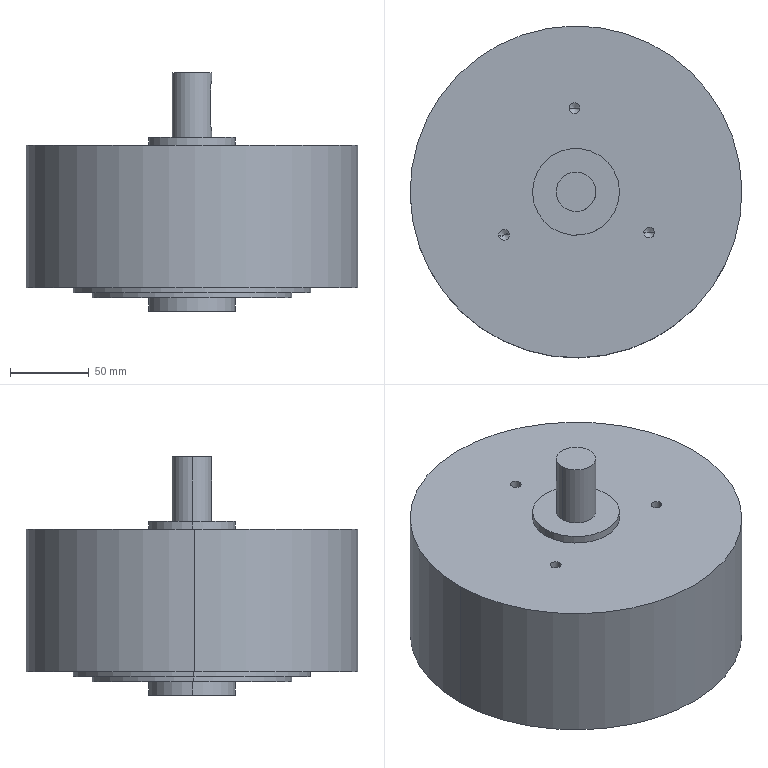Component | SolidWorks | HB-114BHysteresisClutch-1 | 1 solid | 37 faces | box 210 x 210 x 151 mm | volume 3263911 mm3 | cylinder 21 | plane 10 | cone 6 | commonest cylinder face diameters 6.8 x6 55 x4 8 x3 126.361 x2 150.627 x2 210 x2 25 x2 | material A3
build123d program:
from build123d import *

# Parameters (mm, degrees)
CUT_EXTRUDE1_START    = 12.5
CUT_EXTRUDE1_DEPTH    = 4
M8_TAPPED_HOLE1_D     = 6.8
M8_TAPPED_HOLE1_DEPTH = 19.75
M8_TAPPED_HOLE1_TIP   = 2.043


with BuildPart() as part:
    # Sketch1 → Revolve1 (revolve)
    with BuildSketch(Plane.XY, mode=Mode.PRIVATE) as revolve1_sk:
        Polygon((0, 0), (151, 0), (151, 27.5), (142.307, 27.5), (142.307, 63.181), (139.421, 63.181), (139.421, 75.314), (136, 75.314), (136, 105), (46, 105), (46, 27.5), (41, 27.5), (41, 12.5), (0, 12.5), align=None)
    revolve(revolve1_sk.sketch.rotate(Axis((0, 0, 0), (-1, 0, 0)), 90), axis=Axis((0, 0, 0), (-1, 0, 0)))

    # Sketch2 → Cut-Extrude1 (cut)
    with BuildSketch(Plane.XY.offset(CUT_EXTRUDE1_START)):
        with BuildLine():
            Line((9, 4), (33, 4))
            ThreePointArc((33, 4), (37, 0), (33, -4))
            Line((33, -4), (9, -4))
            ThreePointArc((9, -4), (5, 0), (9, 4))
        make_face()
    extrude(amount=-CUT_EXTRUDE1_DEPTH, mode=Mode.SUBTRACT)

    # M8 Tapped Hole1
    with Locations(Plane.ZY.offset(-46)):
        with Locations((0, 53), (45.899, -26.5), (-45.899, -26.5)):
            Hole(M8_TAPPED_HOLE1_D / 2, depth=M8_TAPPED_HOLE1_DEPTH)
            with Locations((0, 0, -(M8_TAPPED_HOLE1_DEPTH + M8_TAPPED_HOLE1_TIP / 2))):  # 118° drill point
                Cone(0, M8_TAPPED_HOLE1_D / 2, M8_TAPPED_HOLE1_TIP, mode=Mode.SUBTRACT)


solid = part.part

# Placed as in the assembly
solid = solid.moved(Location((733.029, 200.722, -58.5), (-90, 89.057, 90)))
STEP:
#1=CARTESIAN_POINT('',(28.691,9.987,-4.892));
#2=VERTEX_POINT('',#1);
#3=CARTESIAN_POINT('',(28.959,9.991,-4.892));
#4=VERTEX_POINT('',#3);
#5=CARTESIAN_POINT('',(28.825,9.989,-4.892));
#6=DIRECTION('',(-0.,-0.,1.));
#7=DIRECTION('',(0.9999,0.01645,0.));
#8=AXIS2_PLACEMENT_3D('',#5,#6,#7);
#9=CIRCLE('',#8,0.1339);
#10=EDGE_CURVE('',#2,#4,#9,.T.);
#11=ORIENTED_EDGE('',*,*,#10,.F.);
#12=CARTESIAN_POINT('',(28.691,9.987,-4.114));
#13=VERTEX_POINT('',#12);
#14=CARTESIAN_POINT('',(28.691,9.987,-4.114));
#15=DIRECTION('',(-0.,-0.,1.));
#16=VECTOR('',#15,39.37);
#17=LINE('',#14,#16);
#18=EDGE_CURVE('',#2,#13,#17,.T.);
#19=ORIENTED_EDGE('',*,*,#18,.T.);
#20=CARTESIAN_POINT('',(28.959,9.991,-4.114));
#21=VERTEX_POINT('',#20);
#22=CARTESIAN_POINT('',(28.825,9.989,-4.114));
#23=DIRECTION('',(-0.,-0.,1.));
#24=DIRECTION('',(0.9999,0.01645,0.));
#25=AXIS2_PLACEMENT_3D('',#22,#23,#24);
#26=CIRCLE('',#25,0.1339);
#27=EDGE_CURVE('',#13,#21,#26,.T.);
#28=ORIENTED_EDGE('',*,*,#27,.T.);
#29=CARTESIAN_POINT('',(28.959,9.991,-4.114));
#30=DIRECTION('',(-0.,-0.,1.));
#31=VECTOR('',#30,39.37);
#32=LINE('',#29,#31);
#33=EDGE_CURVE('',#4,#21,#32,.T.);
#34=ORIENTED_EDGE('',*,*,#33,.F.);
#35=EDGE_LOOP('',(#11,#19,#28,#34));
#36=FACE_OUTER_BOUND('',#35,.T.);
#37=CARTESIAN_POINT('',(28.825,9.989,-4.114));
#38=DIRECTION('',(-0.,-0.,1.));
#39=DIRECTION('',(0.9999,0.01645,0.));
#40=AXIS2_PLACEMENT_3D('',#37,#38,#39);
#41=CYLINDRICAL_SURFACE('',#40,0.1339);
#42=ADVANCED_FACE('',(#36),#41,.F.);
#43=CARTESIAN_POINT('',(28.825,9.989,-4.972));
#44=VERTEX_POINT('',#43);
#45=CARTESIAN_POINT('',(28.959,9.991,-4.892));
#46=DIRECTION('',(0.8571,0.0141,0.515));
#47=VECTOR('',#46,39.37);
#48=LINE('',#45,#47);
#49=EDGE_CURVE('',#44,#4,#48,.T.);
#50=ORIENTED_EDGE('',*,*,#49,.F.);
#51=CARTESIAN_POINT('',(28.691,9.987,-4.892));
#52=DIRECTION('',(-0.8571,-0.0141,0.515));
#53=VECTOR('',#52,39.37);
#54=LINE('',#51,#53);
#55=EDGE_CURVE('',#44,#2,#54,.T.);
#56=ORIENTED_EDGE('',*,*,#55,.T.);
#57=ORIENTED_EDGE('',*,*,#10,.T.);
#58=EDGE_LOOP('',(#50,#56,#57));
#59=FACE_OUTER_BOUND('',#58,.T.);
#60=CARTESIAN_POINT('',(28.825,9.989,-4.892));
#61=DIRECTION('',(-0.,-0.,1.));
#62=DIRECTION('',(0.9999,0.01645,0.));
#63=AXIS2_PLACEMENT_3D('',#60,#61,#62);
#64=CONICAL_SURFACE('',#63,0.1339,1.03);
#65=ADVANCED_FACE('',(#59),#64,.F.);
#66=CARTESIAN_POINT('',(30.55,6.887,-4.892));
#67=VERTEX_POINT('',#66);
#68=CARTESIAN_POINT('',(30.817,6.891,-4.892));
#69=VERTEX_POINT('',#68);
#70=CARTESIAN_POINT('',(30.683,6.889,-4.892));
#71=DIRECTION('',(-0.,-0.,1.));
#72=DIRECTION('',(0.9999,0.01645,0.));
#73=AXIS2_PLACEMENT_3D('',#70,#71,#72);
#74=CIRCLE('',#73,0.1339);
#75=EDGE_CURVE('',#67,#69,#74,.T.);
#76=ORIENTED_EDGE('',*,*,#75,.F.);
#77=CARTESIAN_POINT('',(30.55,6.887,-4.114));
#78=VERTEX_POINT('',#77);
#79=CARTESIAN_POINT('',(30.55,6.887,-4.114));
#80=DIRECTION('',(-0.,-0.,1.));
#81=VECTOR('',#80,39.37);
#82=LINE('',#79,#81);
#83=EDGE_CURVE('',#67,#78,#82,.T.);
#84=ORIENTED_EDGE('',*,*,#83,.T.);
#85=CARTESIAN_POINT('',(30.817,6.891,-4.114));
#86=VERTEX_POINT('',#85);
#87=CARTESIAN_POINT('',(30.683,6.889,-4.114));
#88=DIRECTION('',(-0.,-0.,1.));
#89=DIRECTION('',(0.9999,0.01645,0.));
#90=AXIS2_PLACEMENT_3D('',#87,#88,#89);
#91=CIRCLE('',#90,0.1339);
#92=EDGE_CURVE('',#78,#86,#91,.T.);
#93=ORIENTED_EDGE('',*,*,#92,.T.);
#94=CARTESIAN_POINT('',(30.817,6.891,-4.114));
#95=DIRECTION('',(-0.,-0.,1.));
#96=VECTOR('',#95,39.37);
#97=LINE('',#94,#96);
#98=EDGE_CURVE('',#69,#86,#97,.T.);
#99=ORIENTED_EDGE('',*,*,#98,.F.);
#100=EDGE_LOOP('',(#76,#84,#93,#99));
#101=FACE_OUTER_BOUND('',#100,.T.);
#102=CARTESIAN_POINT('',(30.683,6.889,-4.114));
#103=DIRECTION('',(-0.,-0.,1.));
#104=DIRECTION('',(0.9999,0.01645,0.));
#105=AXIS2_PLACEMENT_3D('',#102,#103,#104);
#106=CYLINDRICAL_SURFACE('',#105,0.1339);
#107=ADVANCED_FACE('',(#101),#106,.F.);
#108=CARTESIAN_POINT('',(30.683,6.889,-4.972));
#109=VERTEX_POINT('',#108);
#110=CARTESIAN_POINT('',(30.817,6.891,-4.892));
#111=DIRECTION('',(0.8571,0.0141,0.515));
#112=VECTOR('',#111,39.37);
#113=LINE('',#110,#112);
#114=EDGE_CURVE('',#109,#69,#113,.T.);
#115=ORIENTED_EDGE('',*,*,#114,.F.);
#116=CARTESIAN_POINT('',(30.55,6.887,-4.892));
#117=DIRECTION('',(-0.8571,-0.0141,0.515));
#118=VECTOR('',#117,39.37);
#119=LINE('',#116,#118);
#120=EDGE_CURVE('',#109,#67,#119,.T.);
#121=ORIENTED_EDGE('',*,*,#120,.T.);
#122=ORIENTED_EDGE('',*,*,#75,.T.);
#123=EDGE_LOOP('',(#115,#121,#122));
#124=FACE_OUTER_BOUND('',#123,.T.);
#125=CARTESIAN_POINT('',(30.683,6.889,-4.892));
#126=DIRECTION('',(-0.,-0.,1.));
#127=DIRECTION('',(0.9999,0.01645,0.));
#128=AXIS2_PLACEMENT_3D('',#125,#126,#127);
#129=CONICAL_SURFACE('',#128,0.1339,1.03);
#130=ADVANCED_FACE('',(#124),#129,.F.);
#131=CARTESIAN_POINT('',(26.936,6.827,-4.892));
#132=VERTEX_POINT('',#131);
#133=CARTESIAN_POINT('',(27.204,6.832,-4.892));
#134=VERTEX_POINT('',#133);
#135=CARTESIAN_POINT('',(27.07,6.83,-4.892));
#136=DIRECTION('',(-0.,-0.,1.));
#137=DIRECTION('',(0.9999,0.01645,0.));
#138=AXIS2_PLACEMENT_3D('',#135,#136,#137);
#139=CIRCLE('',#138,0.1339);
#140=EDGE_CURVE('',#132,#134,#139,.T.);
#141=ORIENTED_EDGE('',*,*,#140,.F.);
#142=CARTESIAN_POINT('',(26.936,6.827,-4.114));
#143=VERTEX_POINT('',#142);
#144=CARTESIAN_POINT('',(26.936,6.827,-4.114));
#145=DIRECTION('',(-0.,-0.,1.));
#146=VECTOR('',#145,39.37);
#147=LINE('',#144,#146);
#148=EDGE_CURVE('',#132,#143,#147,.T.);
#149=ORIENTED_EDGE('',*,*,#148,.T.);
#150=CARTESIAN_POINT('',(27.204,6.832,-4.114));
#151=VERTEX_POINT('',#150);
#152=CARTESIAN_POINT('',(27.07,6.83,-4.114));
#153=DIRECTION('',(-0.,-0.,1.));
#154=DIRECTION('',(0.9999,0.01645,0.));
#155=AXIS2_PLACEMENT_3D('',#152,#153,#154);
#156=CIRCLE('',#155,0.1339);
#157=EDGE_CURVE('',#143,#151,#156,.T.);
#158=ORIENTED_EDGE('',*,*,#157,.T.);
#159=CARTESIAN_POINT('',(27.204,6.832,-4.114));
#160=DIRECTION('',(-0.,-0.,1.));
#161=VECTOR('',#160,39.37);
#162=LINE('',#159,#161);
#163=EDGE_CURVE('',#134,#151,#162,.T.);
#164=ORIENTED_EDGE('',*,*,#163,.F.);
#165=EDGE_LOOP('',(#141,#149,#158,#164));
#166=FACE_OUTER_BOUND('',#165,.T.);
#167=CARTESIAN_POINT('',(27.07,6.83,-4.114));
#168=DIRECTION('',(-0.,-0.,1.));
#169=DIRECTION('',(0.9999,0.01645,0.));
#170=AXIS2_PLACEMENT_3D('',#167,#168,#169);
#171=CYLINDRICAL_SURFACE('',#170,0.1339);
#172=ADVANCED_FACE('',(#166),#171,.F.);
#173=CARTESIAN_POINT('',(27.07,6.83,-4.972));
#174=VERTEX_POINT('',#173);
#175=CARTESIAN_POINT('',(27.204,6.832,-4.892));
#176=DIRECTION('',(0.8571,0.0141,0.515));
#177=VECTOR('',#176,39.37);
#178=LINE('',#175,#177);
#179=EDGE_CURVE('',#174,#134,#178,.T.);
#180=ORIENTED_EDGE('',*,*,#179,.F.);
#181=CARTESIAN_POINT('',(26.936,6.827,-4.892));
#182=DIRECTION('',(-0.8571,-0.0141,0.515));
#183=VECTOR('',#182,39.37);
#184=LINE('',#181,#183);
#185=EDGE_CURVE('',#174,#132,#184,.T.);
#186=ORIENTED_EDGE('',*,*,#185,.T.);
#187=ORIENTED_EDGE('',*,*,#140,.T.);
#188=EDGE_LOOP('',(#180,#186,#187));
#189=FACE_OUTER_BOUND('',#188,.T.);
#190=CARTESIAN_POINT('',(27.07,6.83,-4.892));
#191=DIRECTION('',(-0.,-0.,1.));
#192=DIRECTION('',(0.9999,0.01645,0.));
#193=AXIS2_PLACEMENT_3D('',#190,#191,#192);
#194=CONICAL_SURFACE('',#193,0.1339,1.03);
#195=ADVANCED_FACE('',(#189),#194,.F.);
#196=CARTESIAN_POINT('',(29.194,7.908,-3.76));
#197=VERTEX_POINT('',#196);
#198=CARTESIAN_POINT('',(29.191,8.065,-3.602));
#199=VERTEX_POINT('',#198);
#200=CARTESIAN_POINT('',(29.194,7.908,-3.602));
#201=DIRECTION('',(0.9999,0.01645,0.));
#202=DIRECTION('',(0.,0.,-1.));
#203=AXIS2_PLACEMENT_3D('',#200,#201,#202);
#204=CIRCLE('',#203,0.1575);
#205=EDGE_CURVE('',#197,#199,#204,.T.);
#206=ORIENTED_EDGE('',*,*,#205,.F.);
#207=CARTESIAN_POINT('',(29.351,7.911,-3.76));
#208=VERTEX_POINT('',#207);
#209=CARTESIAN_POINT('',(29.194,7.908,-3.76));
#210=DIRECTION('',(0.9999,0.01645,0.));
#211=VECTOR('',#210,39.37);
#212=LINE('',#209,#211);
#213=EDGE_CURVE('',#197,#208,#212,.T.);
#214=ORIENTED_EDGE('',*,*,#213,.T.);
#215=CARTESIAN_POINT('',(29.323,8.068,-3.602));
#216=VERTEX_POINT('',#215);
#217=CARTESIAN_POINT('',(29.351,7.911,-3.76));
#218=CARTESIAN_POINT('',(29.351,7.921,-3.76));
#219=CARTESIAN_POINT('',(29.351,7.931,-3.759));
#220=CARTESIAN_POINT('',(29.349,7.952,-3.755));
#221=CARTESIAN_POINT('',(29.348,7.961,-3.752));
#222=CARTESIAN_POINT('',(29.345,7.981,-3.744));
#223=CARTESIAN_POINT('',(29.344,7.99,-3.739));
#224=CARTESIAN_POINT('',(29.34,8.006,-3.728));
#225=CARTESIAN_POINT('',(29.339,8.014,-3.721));
#226=CARTESIAN_POINT('',(29.335,8.029,-3.706));
#227=CARTESIAN_POINT('',(29.333,8.035,-3.699));
#228=CARTESIAN_POINT('',(29.33,8.047,-3.682));
#229=CARTESIAN_POINT('',(29.328,8.052,-3.672));
#230=CARTESIAN_POINT('',(29.326,8.059,-3.653));
#231=CARTESIAN_POINT('',(29.325,8.062,-3.644));
#232=CARTESIAN_POINT('',(29.323,8.067,-3.623));
#233=CARTESIAN_POINT('',(29.323,8.068,-3.613));
#234=CARTESIAN_POINT('',(29.323,8.068,-3.602));
#235=B_SPLINE_CURVE_WITH_KNOTS('',3,(#217,#218,#219,#220,#221,#222,#223,#224,#225,#226,#227,#228,#229,#230,#231,#232,#233,#234),.UNSPECIFIED.,.F.,.F.,(4,2,2,2,2,2,2,2,4),(0.006296,0.007082,0.007868,0.008654,0.00944,0.01023,0.01101,0.0118,0.01258),.UNSPECIFIED.);
#236=EDGE_CURVE('',#208,#216,#235,.T.);
#237=ORIENTED_EDGE('',*,*,#236,.T.);
#238=CARTESIAN_POINT('',(29.191,8.065,-3.602));
#239=DIRECTION('',(0.9999,0.01645,0.));
#240=VECTOR('',#239,39.37);
#241=LINE('',#238,#240);
#242=EDGE_CURVE('',#199,#216,#241,.T.);
#243=ORIENTED_EDGE('',*,*,#242,.F.);
#244=EDGE_LOOP('',(#206,#214,#237,#243));
#245=FACE_OUTER_BOUND('',#244,.T.);
#246=CARTESIAN_POINT('',(29.194,7.908,-3.602));
#247=DIRECTION('',(0.9999,0.01645,0.));
#248=DIRECTION('',(0.,0.,-1.));
#249=AXIS2_PLACEMENT_3D('',#246,#247,#248);
#250=CYLINDRICAL_SURFACE('',#249,0.1575);
#251=ADVANCED_FACE('',(#245),#250,.F.);
#252=CARTESIAN_POINT('',(26.372,7.862,-7.792));
#253=VERTEX_POINT('',#252);
#254=CARTESIAN_POINT('',(31.346,7.943,-7.792));
#255=VERTEX_POINT('',#254);
#256=CARTESIAN_POINT('',(28.859,7.902,-7.792));
#257=DIRECTION('',(0.,0.,-1.));
#258=DIRECTION('',(-0.9999,-0.01645,0.));
#259=AXIS2_PLACEMENT_3D('',#256,#257,#258);
#260=CIRCLE('',#259,2.487);
#261=EDGE_CURVE('',#253,#255,#260,.T.);
#262=ORIENTED_EDGE('',*,*,#261,.T.);
#263=CARTESIAN_POINT('',(31.346,7.943,-7.906));
#264=VERTEX_POINT('',#263);
#265=CARTESIAN_POINT('',(31.346,7.943,-2.303));
#266=DIRECTION('',(0.,0.,-1.));
#267=VECTOR('',#266,39.37);
#268=LINE('',#265,#267);
#269=EDGE_CURVE('',#255,#264,#268,.T.);
#270=ORIENTED_EDGE('',*,*,#269,.T.);
#271=CARTESIAN_POINT('',(26.372,7.862,-7.906));
#272=VERTEX_POINT('',#271);
#273=CARTESIAN_POINT('',(28.859,7.902,-7.906));
#274=DIRECTION('',(0.,0.,-1.));
#275=DIRECTION('',(-0.9999,-0.01645,0.));
#276=AXIS2_PLACEMENT_3D('',#273,#274,#275);
#277=CIRCLE('',#276,2.487);
#278=EDGE_CURVE('',#272,#264,#277,.T.);
#279=ORIENTED_EDGE('',*,*,#278,.F.);
#280=CARTESIAN_POINT('',(26.372,7.862,-2.303));
#281=DIRECTION('',(0.,0.,-1.));
#282=VECTOR('',#281,39.37);
#283=LINE('',#280,#282);
#284=EDGE_CURVE('',#253,#272,#283,.T.);
#285=ORIENTED_EDGE('',*,*,#284,.F.);
#286=EDGE_LOOP('',(#262,#270,#279,#285));
#287=FACE_OUTER_BOUND('',#286,.T.);
#288=CARTESIAN_POINT('',(28.859,7.902,-2.303));
#289=DIRECTION('',(0.,0.,-1.));
#290=DIRECTION('',(-0.9999,-0.01645,0.));
#291=AXIS2_PLACEMENT_3D('',#288,#289,#290);
#292=CYLINDRICAL_SURFACE('',#291,2.487);
#293=ADVANCED_FACE('',(#287),#292,.T.);
#294=CARTESIAN_POINT('',(25.895,7.854,-7.657));
#295=VERTEX_POINT('',#294);
#296=CARTESIAN_POINT('',(31.824,7.951,-7.657));
#297=VERTEX_POINT('',#296);
#298=CARTESIAN_POINT('',(28.859,7.902,-7.657));
#299=DIRECTION('',(0.,0.,-1.));
#300=DIRECTION('',(-0.9999,-0.01645,0.));
#301=AXIS2_PLACEMENT_3D('',#298,#299,#300);
#302=CIRCLE('',#301,2.965);
#303=EDGE_CURVE('',#295,#297,#302,.T.);
#304=ORIENTED_EDGE('',*,*,#303,.T.);
#305=CARTESIAN_POINT('',(31.824,7.951,-7.792));
#306=VERTEX_POINT('',#305);
#307=CARTESIAN_POINT('',(31.824,7.951,-2.303));
#308=DIRECTION('',(0.,0.,-1.));
#309=VECTOR('',#308,39.37);
#310=LINE('',#307,#309);
#311=EDGE_CURVE('',#297,#306,#310,.T.);
#312=ORIENTED_EDGE('',*,*,#311,.T.);
#313=CARTESIAN_POINT('',(25.895,7.854,-7.792));
#314=VERTEX_POINT('',#313);
#315=CARTESIAN_POINT('',(28.859,7.902,-7.792));
#316=DIRECTION('',(0.,0.,-1.));
#317=DIRECTION('',(-0.9999,-0.01645,0.));
#318=AXIS2_PLACEMENT_3D('',#315,#316,#317);
#319=CIRCLE('',#318,2.965);
#320=EDGE_CURVE('',#314,#306,#319,.T.);
#321=ORIENTED_EDGE('',*,*,#320,.F.);
#322=CARTESIAN_POINT('',(25.895,7.854,-2.303));
#323=DIRECTION('',(0.,0.,-1.));
#324=VECTOR('',#323,39.37);
#325=LINE('',#322,#324);
#326=EDGE_CURVE('',#295,#314,#325,.T.);
#327=ORIENTED_EDGE('',*,*,#326,.F.);
#328=EDGE_LOOP('',(#304,#312,#321,#327));
#329=FACE_OUTER_BOUND('',#328,.T.);
#330=CARTESIAN_POINT('',(28.859,7.902,-2.303));
#331=DIRECTION('',(0.,0.,-1.));
#332=DIRECTION('',(-0.9999,-0.01645,0.));
#333=AXIS2_PLACEMENT_3D('',#330,#331,#332);
#334=CYLINDRICAL_SURFACE('',#333,2.965);
#335=ADVANCED_FACE('',(#329),#334,.T.);
#336=CARTESIAN_POINT('',(24.726,7.834,-4.114));
#337=VERTEX_POINT('',#336);
#338=CARTESIAN_POINT('',(32.993,7.97,-4.114));
#339=VERTEX_POINT('',#338);
#340=CARTESIAN_POINT('',(28.859,7.902,-4.114));
#341=DIRECTION('',(0.,0.,-1.));
#342=DIRECTION('',(-0.9999,-0.01645,0.));
#343=AXIS2_PLACEMENT_3D('',#340,#341,#342);
#344=CIRCLE('',#343,4.134);
#345=EDGE_CURVE('',#337,#339,#344,.T.);
#346=ORIENTED_EDGE('',*,*,#345,.T.);
#347=CARTESIAN_POINT('',(32.993,7.97,-7.657));
#348=VERTEX_POINT('',#347);
#349=CARTESIAN_POINT('',(32.993,7.97,-2.303));
#350=DIRECTION('',(0.,0.,-1.));
#351=VECTOR('',#350,39.37);
#352=LINE('',#349,#351);
#353=EDGE_CURVE('',#339,#348,#352,.T.);
#354=ORIENTED_EDGE('',*,*,#353,.T.);
#355=CARTESIAN_POINT('',(24.726,7.834,-7.657));
#356=VERTEX_POINT('',#355);
#357=CARTESIAN_POINT('',(28.859,7.902,-7.657));
#358=DIRECTION('',(0.,0.,-1.));
#359=DIRECTION('',(-0.9999,-0.01645,0.));
#360=AXIS2_PLACEMENT_3D('',#357,#358,#359);
#361=CIRCLE('',#360,4.134);
#362=EDGE_CURVE('',#356,#348,#361,.T.);
#363=ORIENTED_EDGE('',*,*,#362,.F.);
#364=CARTESIAN_POINT('',(24.726,7.834,-2.303));
#365=DIRECTION('',(0.,0.,-1.));
#366=VECTOR('',#365,39.37);
#367=LINE('',#364,#366);
#368=EDGE_CURVE('',#337,#356,#367,.T.);
#369=ORIENTED_EDGE('',*,*,#368,.F.);
#370=EDGE_LOOP('',(#346,#354,#363,#369));
#371=FACE_OUTER_BOUND('',#370,.T.);
#372=CARTESIAN_POINT('',(28.859,7.902,-2.303));
#373=DIRECTION('',(0.,0.,-1.));
#374=DIRECTION('',(-0.9999,-0.01645,0.));
#375=AXIS2_PLACEMENT_3D('',#372,#373,#374);
#376=CYLINDRICAL_SURFACE('',#375,4.134);
#377=ADVANCED_FACE('',(#371),#376,.T.);
#378=CARTESIAN_POINT('',(27.777,7.885,-3.917));
#379=VERTEX_POINT('',#378);
#380=CARTESIAN_POINT('',(29.942,7.92,-3.917));
#381=VERTEX_POINT('',#380);
#382=CARTESIAN_POINT('',(28.859,7.902,-3.917));
#383=DIRECTION('',(0.,0.,-1.));
#384=DIRECTION('',(-0.9999,-0.01645,0.));
#385=AXIS2_PLACEMENT_3D('',#382,#383,#384);
#386=CIRCLE('',#385,1.083);
#387=EDGE_CURVE('',#379,#381,#386,.T.);
#388=ORIENTED_EDGE('',*,*,#387,.T.);
#389=CARTESIAN_POINT('',(29.942,7.92,-4.114));
#390=VERTEX_POINT('',#389);
#391=CARTESIAN_POINT('',(29.942,7.92,-2.303));
#392=DIRECTION('',(0.,0.,-1.));
#393=VECTOR('',#392,39.37);
#394=LINE('',#391,#393);
#395=EDGE_CURVE('',#381,#390,#394,.T.);
#396=ORIENTED_EDGE('',*,*,#395,.T.);
#397=CARTESIAN_POINT('',(27.777,7.885,-4.114));
#398=VERTEX_POINT('',#397);
#399=CARTESIAN_POINT('',(28.859,7.902,-4.114));
#400=DIRECTION('',(0.,0.,-1.));
#401=DIRECTION('',(-0.9999,-0.01645,0.));
#402=AXIS2_PLACEMENT_3D('',#399,#400,#401);
#403=CIRCLE('',#402,1.083);
#404=EDGE_CURVE('',#398,#390,#403,.T.);
#405=ORIENTED_EDGE('',*,*,#404,.F.);
#406=CARTESIAN_POINT('',(27.777,7.885,-2.303));
#407=DIRECTION('',(0.,0.,-1.));
#408=VECTOR('',#407,39.37);
#409=LINE('',#406,#408);
#410=EDGE_CURVE('',#379,#398,#409,.T.);
#411=ORIENTED_EDGE('',*,*,#410,.F.);
#412=EDGE_LOOP('',(#388,#396,#405,#411));
#413=FACE_OUTER_BOUND('',#412,.T.);
#414=CARTESIAN_POINT('',(28.859,7.902,-2.303));
#415=DIRECTION('',(0.,0.,-1.));
#416=DIRECTION('',(-0.9999,-0.01645,0.));
#417=AXIS2_PLACEMENT_3D('',#414,#415,#416);
#418=CYLINDRICAL_SURFACE('',#417,1.083);
#419=ADVANCED_FACE('',(#413),#418,.T.);
#420=CARTESIAN_POINT('',(28.367,7.894,-2.303));
#421=VERTEX_POINT('',#420);
#422=CARTESIAN_POINT('',(29.351,7.911,-2.303));
#423=VERTEX_POINT('',#422);
#424=CARTESIAN_POINT('',(28.859,7.902,-2.303));
#425=DIRECTION('',(0.,0.,-1.));
#426=DIRECTION('',(-0.9999,-0.01645,0.));
#427=AXIS2_PLACEMENT_3D('',#424,#425,#426);
#428=CIRCLE('',#427,0.4921);
#429=EDGE_CURVE('',#421,#423,#428,.T.);
#430=ORIENTED_EDGE('',*,*,#429,.T.);
#431=CARTESIAN_POINT('',(29.351,7.911,-2.5));
#432=VERTEX_POINT('',#431);
#433=CARTESIAN_POINT('',(29.351,7.911,-2.303));
#434=DIRECTION('',(0.,0.,-1.));
#435=VECTOR('',#434,39.37);
#436=LINE('',#433,#435);
#437=EDGE_CURVE('',#423,#432,#436,.T.);
#438=ORIENTED_EDGE('',*,*,#437,.T.);
#439=CARTESIAN_POINT('',(29.323,8.068,-2.657));
#440=VERTEX_POINT('',#439);
#441=CARTESIAN_POINT('',(29.323,8.068,-2.657));
#442=CARTESIAN_POINT('',(29.323,8.068,-2.647));
#443=CARTESIAN_POINT('',(29.323,8.067,-2.637));
#444=CARTESIAN_POINT('',(29.325,8.063,-2.616));
#445=CARTESIAN_POINT('',(29.326,8.059,-2.606));
#446=CARTESIAN_POINT('',(29.328,8.052,-2.587));
#447=CARTESIAN_POINT('',(29.33,8.047,-2.578));
#448=CARTESIAN_POINT('',(29.333,8.035,-2.561));
#449=CARTESIAN_POINT('',(29.335,8.029,-2.553));
#450=CARTESIAN_POINT('',(29.339,8.014,-2.539));
#451=CARTESIAN_POINT('',(29.34,8.007,-2.532));
#452=CARTESIAN_POINT('',(29.344,7.989,-2.521));
#453=CARTESIAN_POINT('',(29.345,7.98,-2.516));
#454=CARTESIAN_POINT('',(29.348,7.961,-2.508));
#455=CARTESIAN_POINT('',(29.349,7.951,-2.505));
#456=CARTESIAN_POINT('',(29.351,7.931,-2.501));
#457=CARTESIAN_POINT('',(29.351,7.921,-2.5));
#458=CARTESIAN_POINT('',(29.351,7.911,-2.5));
#459=B_SPLINE_CURVE_WITH_KNOTS('',3,(#441,#442,#443,#444,#445,#446,#447,#448,#449,#450,#451,#452,#453,#454,#455,#456,#457,#458),.UNSPECIFIED.,.F.,.F.,(4,2,2,2,2,2,2,2,4),(0.,0.000787,0.001574,0.002361,0.003148,0.003935,0.004722,0.005509,0.006296),.UNSPECIFIED.);
#460=EDGE_CURVE('',#440,#432,#459,.T.);
#461=ORIENTED_EDGE('',*,*,#460,.F.);
#462=CARTESIAN_POINT('',(29.323,8.068,-2.303));
#463=DIRECTION('',(-0.,-0.,1.));
#464=VECTOR('',#463,39.37);
#465=LINE('',#462,#464);
#466=EDGE_CURVE('',#216,#440,#465,.T.);
#467=ORIENTED_EDGE('',*,*,#466,.F.);
#468=ORIENTED_EDGE('',*,*,#236,.F.);
#469=CARTESIAN_POINT('',(29.351,7.911,-3.917));
#470=VERTEX_POINT('',#469);
#471=CARTESIAN_POINT('',(29.351,7.911,-2.303));
#472=DIRECTION('',(0.,0.,-1.));
#473=VECTOR('',#472,39.37);
#474=LINE('',#471,#473);
#475=EDGE_CURVE('',#208,#470,#474,.T.);
#476=ORIENTED_EDGE('',*,*,#475,.T.);
#477=CARTESIAN_POINT('',(28.367,7.894,-3.917));
#478=VERTEX_POINT('',#477);
#479=CARTESIAN_POINT('',(28.859,7.902,-3.917));
#480=DIRECTION('',(0.,0.,-1.));
#481=DIRECTION('',(-0.9999,-0.01645,0.));
#482=AXIS2_PLACEMENT_3D('',#479,#480,#481);
#483=CIRCLE('',#482,0.4921);
#484=EDGE_CURVE('',#478,#470,#483,.T.);
#485=ORIENTED_EDGE('',*,*,#484,.F.);
#486=CARTESIAN_POINT('',(28.367,7.894,-2.303));
#487=DIRECTION('',(0.,0.,-1.));
#488=VECTOR('',#487,39.37);
#489=LINE('',#486,#488);
#490=EDGE_CURVE('',#421,#478,#489,.T.);
#491=ORIENTED_EDGE('',*,*,#490,.F.);
#492=EDGE_LOOP('',(#430,#438,#461,#467,#468,#476,#485,#491));
#493=FACE_OUTER_BOUND('',#492,.T.);
#494=CARTESIAN_POINT('',(28.859,7.902,-2.303));
#495=DIRECTION('',(0.,0.,-1.));
#496=DIRECTION('',(-0.9999,-0.01645,0.));
#497=AXIS2_PLACEMENT_3D('',#494,#495,#496);
#498=CYLINDRICAL_SURFACE('',#497,0.4921);
#499=ADVANCED_FACE('',(#493),#498,.T.);
#500=CARTESIAN_POINT('',(27.777,7.885,-7.906));
#501=VERTEX_POINT('',#500);
#502=CARTESIAN_POINT('',(29.942,7.92,-7.906));
#503=VERTEX_POINT('',#502);
#504=CARTESIAN_POINT('',(28.859,7.902,-7.906));
#505=DIRECTION('',(0.,0.,-1.));
#506=DIRECTION('',(-0.9999,-0.01645,0.));
#507=AXIS2_PLACEMENT_3D('',#504,#505,#506);
#508=CIRCLE('',#507,1.083);
#509=EDGE_CURVE('',#501,#503,#508,.T.);
#510=ORIENTED_EDGE('',*,*,#509,.T.);
#511=CARTESIAN_POINT('',(29.942,7.92,-8.248));
#512=VERTEX_POINT('',#511);
#513=CARTESIAN_POINT('',(29.942,7.92,-2.303));
#514=DIRECTION('',(0.,0.,-1.));
#515=VECTOR('',#514,39.37);
#516=LINE('',#513,#515);
#517=EDGE_CURVE('',#503,#512,#516,.T.);
#518=ORIENTED_EDGE('',*,*,#517,.T.);
#519=CARTESIAN_POINT('',(27.777,7.885,-8.248));
#520=VERTEX_POINT('',#519);
#521=CARTESIAN_POINT('',(28.859,7.902,-8.248));
#522=DIRECTION('',(0.,0.,-1.));
#523=DIRECTION('',(-0.9999,-0.01645,0.));
#524=AXIS2_PLACEMENT_3D('',#521,#522,#523);
#525=CIRCLE('',#524,1.083);
#526=EDGE_CURVE('',#520,#512,#525,.T.);
#527=ORIENTED_EDGE('',*,*,#526,.F.);
#528=CARTESIAN_POINT('',(27.777,7.885,-2.303));
#529=DIRECTION('',(0.,0.,-1.));
#530=VECTOR('',#529,39.37);
#531=LINE('',#528,#530);
#532=EDGE_CURVE('',#501,#520,#531,.T.);
#533=ORIENTED_EDGE('',*,*,#532,.F.);
#534=EDGE_LOOP('',(#510,#518,#527,#533));
#535=FACE_OUTER_BOUND('',#534,.T.);
#536=CARTESIAN_POINT('',(28.859,7.902,-2.303));
#537=DIRECTION('',(0.,0.,-1.));
#538=DIRECTION('',(-0.9999,-0.01645,0.));
#539=AXIS2_PLACEMENT_3D('',#536,#537,#538);
#540=CYLINDRICAL_SURFACE('',#539,1.083);
#541=ADVANCED_FACE('',(#535),#540,.T.);
#542=ORIENTED_EDGE('',*,*,#517,.F.);
#543=CARTESIAN_POINT('',(28.859,7.902,-7.906));
#544=DIRECTION('',(0.,0.,-1.));
#545=DIRECTION('',(-0.9999,-0.01645,0.));
#546=AXIS2_PLACEMENT_3D('',#543,#544,#545);
#547=CIRCLE('',#546,1.083);
#548=EDGE_CURVE('',#503,#501,#547,.T.);
#549=ORIENTED_EDGE('',*,*,#548,.T.);
#550=ORIENTED_EDGE('',*,*,#532,.T.);
#551=CARTESIAN_POINT('',(28.859,7.902,-8.248));
#552=DIRECTION('',(0.,0.,-1.));
#553=DIRECTION('',(-0.9999,-0.01645,0.));
#554=AXIS2_PLACEMENT_3D('',#551,#552,#553);
#555=CIRCLE('',#554,1.083);
#556=EDGE_CURVE('',#512,#520,#555,.T.);
#557=ORIENTED_EDGE('',*,*,#556,.F.);
#558=EDGE_LOOP('',(#542,#549,#550,#557));
#559=FACE_OUTER_BOUND('',#558,.T.);
#560=CARTESIAN_POINT('',(28.859,7.902,-2.303));
#561=DIRECTION('',(0.,0.,-1.));
#562=DIRECTION('',(-0.9999,-0.01645,0.));
#563=AXIS2_PLACEMENT_3D('',#560,#561,#562);
#564=CYLINDRICAL_SURFACE('',#563,1.083);
#565=ADVANCED_FACE('',(#559),#564,.T.);
#566=ORIENTED_EDGE('',*,*,#526,.T.);
#567=ORIENTED_EDGE('',*,*,#556,.T.);
#568=EDGE_LOOP('',(#566,#567));
#569=FACE_OUTER_BOUND('',#568,.T.);
#570=CARTESIAN_POINT('',(28.859,7.902,-8.248));
#571=DIRECTION('',(0.,0.,-1.));
#572=DIRECTION('',(-0.9999,-0.01645,-0.));
#573=AXIS2_PLACEMENT_3D('',#570,#571,#572);
#574=PLANE('',#573);
#575=ADVANCED_FACE('',(#569),#574,.T.);
#576=ORIENTED_EDGE('',*,*,#429,.F.);
#577=CARTESIAN_POINT('',(28.859,7.902,-2.303));
#578=DIRECTION('',(0.,0.,-1.));
#579=DIRECTION('',(-0.9999,-0.01645,0.));
#580=AXIS2_PLACEMENT_3D('',#577,#578,#579);
#581=CIRCLE('',#580,0.4921);
#582=EDGE_CURVE('',#423,#421,#581,.T.);
#583=ORIENTED_EDGE('',*,*,#582,.F.);
#584=EDGE_LOOP('',(#576,#583));
#585=FACE_OUTER_BOUND('',#584,.T.);
#586=CARTESIAN_POINT('',(28.851,8.394,-2.303));
#587=DIRECTION('',(-0.,-0.,1.));
#588=DIRECTION('',(0.9999,0.01645,0.));
#589=AXIS2_PLACEMENT_3D('',#586,#587,#588);
#590=PLANE('',#589);
#591=ADVANCED_FACE('',(#585),#590,.T.);
#592=ORIENTED_EDGE('',*,*,#437,.F.);
#593=ORIENTED_EDGE('',*,*,#582,.T.);
#594=ORIENTED_EDGE('',*,*,#490,.T.);
#595=CARTESIAN_POINT('',(28.859,7.902,-3.917));
#596=DIRECTION('',(0.,0.,-1.));
#597=DIRECTION('',(-0.9999,-0.01645,0.));
#598=AXIS2_PLACEMENT_3D('',#595,#596,#597);
#599=CIRCLE('',#598,0.4921);
#600=EDGE_CURVE('',#470,#478,#599,.T.);
#601=ORIENTED_EDGE('',*,*,#600,.F.);
#602=ORIENTED_EDGE('',*,*,#475,.F.);
#603=CARTESIAN_POINT('',(29.328,7.753,-3.602));
#604=VERTEX_POINT('',#603);
#605=CARTESIAN_POINT('',(29.328,7.753,-3.602));
#606=CARTESIAN_POINT('',(29.328,7.753,-3.613));
#607=CARTESIAN_POINT('',(29.329,7.754,-3.623));
#608=CARTESIAN_POINT('',(29.33,7.758,-3.643));
#609=CARTESIAN_POINT('',(29.331,7.761,-3.653));
#610=CARTESIAN_POINT('',(29.333,7.769,-3.672));
#611=CARTESIAN_POINT('',(29.334,7.774,-3.681));
#612=CARTESIAN_POINT('',(29.337,7.785,-3.699));
#613=CARTESIAN_POINT('',(29.339,7.792,-3.707));
#614=CARTESIAN_POINT('',(29.342,7.806,-3.721));
#615=CARTESIAN_POINT('',(29.344,7.814,-3.727));
#616=CARTESIAN_POINT('',(29.346,7.831,-3.739));
#617=CARTESIAN_POINT('',(29.348,7.841,-3.744));
#618=CARTESIAN_POINT('',(29.35,7.859,-3.752));
#619=CARTESIAN_POINT('',(29.351,7.87,-3.755));
#620=CARTESIAN_POINT('',(29.351,7.89,-3.759));
#621=CARTESIAN_POINT('',(29.352,7.9,-3.76));
#622=CARTESIAN_POINT('',(29.351,7.911,-3.76));
#623=B_SPLINE_CURVE_WITH_KNOTS('',3,(#605,#606,#607,#608,#609,#610,#611,#612,#613,#614,#615,#616,#617,#618,#619,#620,#621,#622),.UNSPECIFIED.,.F.,.F.,(4,2,2,2,2,2,2,2,4),(0.,0.000787,0.001574,0.002361,0.003148,0.003935,0.004722,0.005509,0.006296),.UNSPECIFIED.);
#624=EDGE_CURVE('',#604,#208,#623,.T.);
#625=ORIENTED_EDGE('',*,*,#624,.F.);
#626=CARTESIAN_POINT('',(29.328,7.753,-2.657));
#627=VERTEX_POINT('',#626);
#628=CARTESIAN_POINT('',(29.328,7.753,-2.303));
#629=DIRECTION('',(0.,0.,-1.));
#630=VECTOR('',#629,39.37);
#631=LINE('',#628,#630);
#632=EDGE_CURVE('',#627,#604,#631,.T.);
#633=ORIENTED_EDGE('',*,*,#632,.F.);
#634=CARTESIAN_POINT('',(29.351,7.911,-2.5));
#635=CARTESIAN_POINT('',(29.352,7.9,-2.5));
#636=CARTESIAN_POINT('',(29.351,7.89,-2.501));
#637=CARTESIAN_POINT('',(29.351,7.869,-2.505));
#638=CARTESIAN_POINT('',(29.35,7.86,-2.508));
#639=CARTESIAN_POINT('',(29.348,7.84,-2.516));
#640=CARTESIAN_POINT('',(29.346,7.831,-2.521));
#641=CARTESIAN_POINT('',(29.344,7.814,-2.532));
#642=CARTESIAN_POINT('',(29.342,7.806,-2.539));
#643=CARTESIAN_POINT('',(29.339,7.792,-2.553));
#644=CARTESIAN_POINT('',(29.337,7.785,-2.561));
#645=CARTESIAN_POINT('',(29.334,7.774,-2.578));
#646=CARTESIAN_POINT('',(29.333,7.769,-2.587));
#647=CARTESIAN_POINT('',(29.331,7.761,-2.606));
#648=CARTESIAN_POINT('',(29.33,7.758,-2.616));
#649=CARTESIAN_POINT('',(29.329,7.754,-2.637));
#650=CARTESIAN_POINT('',(29.328,7.753,-2.647));
#651=CARTESIAN_POINT('',(29.328,7.753,-2.657));
#652=B_SPLINE_CURVE_WITH_KNOTS('',3,(#634,#635,#636,#637,#638,#639,#640,#641,#642,#643,#644,#645,#646,#647,#648,#649,#650,#651),.UNSPECIFIED.,.F.,.F.,(4,2,2,2,2,2,2,2,4),(0.006296,0.007082,0.007868,0.008654,0.00944,0.01023,0.01101,0.0118,0.01258),.UNSPECIFIED.);
#653=EDGE_CURVE('',#432,#627,#652,.T.);
#654=ORIENTED_EDGE('',*,*,#653,.F.);
#655=EDGE_LOOP('',(#592,#593,#594,#601,#602,#625,#633,#654));
#656=FACE_OUTER_BOUND('',#655,.T.);
#657=CARTESIAN_POINT('',(28.859,7.902,-2.303));
#658=DIRECTION('',(0.,0.,-1.));
#659=DIRECTION('',(-0.9999,-0.01645,0.));
#660=AXIS2_PLACEMENT_3D('',#657,#658,#659);
#661=CYLINDRICAL_SURFACE('',#660,0.4921);
#662=ADVANCED_FACE('',(#656),#661,.T.);
#663=ORIENTED_EDGE('',*,*,#484,.T.);
#664=ORIENTED_EDGE('',*,*,#600,.T.);
#665=EDGE_LOOP('',(#663,#664));
#666=FACE_BOUND('',#665,.T.);
#667=ORIENTED_EDGE('',*,*,#387,.F.);
#668=CARTESIAN_POINT('',(28.859,7.902,-3.917));
#669=DIRECTION('',(0.,0.,-1.));
#670=DIRECTION('',(-0.9999,-0.01645,0.));
#671=AXIS2_PLACEMENT_3D('',#668,#669,#670);
#672=CIRCLE('',#671,1.083);
#673=EDGE_CURVE('',#381,#379,#672,.T.);
#674=ORIENTED_EDGE('',*,*,#673,.F.);
#675=EDGE_LOOP('',(#667,#674));
#676=FACE_OUTER_BOUND('',#675,.T.);
#677=CARTESIAN_POINT('',(28.842,8.985,-3.917));
#678=DIRECTION('',(-0.,-0.,1.));
#679=DIRECTION('',(0.9999,0.01645,0.));
#680=AXIS2_PLACEMENT_3D('',#677,#678,#679);
#681=PLANE('',#680);
#682=ADVANCED_FACE('',(#666,#676),#681,.T.);
#683=ORIENTED_EDGE('',*,*,#395,.F.);
#684=ORIENTED_EDGE('',*,*,#673,.T.);
#685=ORIENTED_EDGE('',*,*,#410,.T.);
#686=CARTESIAN_POINT('',(28.859,7.902,-4.114));
#687=DIRECTION('',(0.,0.,-1.));
#688=DIRECTION('',(-0.9999,-0.01645,0.));
#689=AXIS2_PLACEMENT_3D('',#686,#687,#688);
#690=CIRCLE('',#689,1.083);
#691=EDGE_CURVE('',#390,#398,#690,.T.);
#692=ORIENTED_EDGE('',*,*,#691,.F.);
#693=EDGE_LOOP('',(#683,#684,#685,#692));
#694=FACE_OUTER_BOUND('',#693,.T.);
#695=CARTESIAN_POINT('',(28.859,7.902,-2.303));
#696=DIRECTION('',(0.,0.,-1.));
#697=DIRECTION('',(-0.9999,-0.01645,0.));
#698=AXIS2_PLACEMENT_3D('',#695,#696,#697);
#699=CYLINDRICAL_SURFACE('',#698,1.083);
#700=ADVANCED_FACE('',(#694),#699,.T.);
#701=CARTESIAN_POINT('',(28.825,9.989,-4.114));
#702=DIRECTION('',(-0.,-0.,1.));
#703=DIRECTION('',(0.9999,0.01645,0.));
#704=AXIS2_PLACEMENT_3D('',#701,#702,#703);
#705=CIRCLE('',#704,0.1339);
#706=EDGE_CURVE('',#21,#13,#705,.T.);
#707=ORIENTED_EDGE('',*,*,#706,.F.);
#708=ORIENTED_EDGE('',*,*,#27,.F.);
#709=EDGE_LOOP('',(#707,#708));
#710=FACE_BOUND('',#709,.T.);
#711=CARTESIAN_POINT('',(30.683,6.889,-4.114));
#712=DIRECTION('',(-0.,-0.,1.));
#713=DIRECTION('',(0.9999,0.01645,0.));
#714=AXIS2_PLACEMENT_3D('',#711,#712,#713);
#715=CIRCLE('',#714,0.1339);
#716=EDGE_CURVE('',#86,#78,#715,.T.);
#717=ORIENTED_EDGE('',*,*,#716,.F.);
#718=ORIENTED_EDGE('',*,*,#92,.F.);
#719=EDGE_LOOP('',(#717,#718));
#720=FACE_BOUND('',#719,.T.);
#721=CARTESIAN_POINT('',(27.07,6.83,-4.114));
#722=DIRECTION('',(-0.,-0.,1.));
#723=DIRECTION('',(0.9999,0.01645,0.));
#724=AXIS2_PLACEMENT_3D('',#721,#722,#723);
#725=CIRCLE('',#724,0.1339);
#726=EDGE_CURVE('',#151,#143,#725,.T.);
#727=ORIENTED_EDGE('',*,*,#726,.F.);
#728=ORIENTED_EDGE('',*,*,#157,.F.);
#729=EDGE_LOOP('',(#727,#728));
#730=FACE_BOUND('',#729,.T.);
#731=ORIENTED_EDGE('',*,*,#404,.T.);
#732=ORIENTED_EDGE('',*,*,#691,.T.);
#733=EDGE_LOOP('',(#731,#732));
#734=FACE_BOUND('',#733,.T.);
#735=ORIENTED_EDGE('',*,*,#345,.F.);
#736=CARTESIAN_POINT('',(28.859,7.902,-4.114));
#737=DIRECTION('',(0.,0.,-1.));
#738=DIRECTION('',(-0.9999,-0.01645,0.));
#739=AXIS2_PLACEMENT_3D('',#736,#737,#738);
#740=CIRCLE('',#739,4.134);
#741=EDGE_CURVE('',#339,#337,#740,.T.);
#742=ORIENTED_EDGE('',*,*,#741,.F.);
#743=EDGE_LOOP('',(#735,#742));
#744=FACE_OUTER_BOUND('',#743,.T.);
#745=CARTESIAN_POINT('',(28.791,12.036,-4.114));
#746=DIRECTION('',(-0.,-0.,1.));
#747=DIRECTION('',(0.9999,0.01645,0.));
#748=AXIS2_PLACEMENT_3D('',#745,#746,#747);
#749=PLANE('',#748);
#750=ADVANCED_FACE('',(#710,#720,#730,#734,#744),#749,.T.);
#751=ORIENTED_EDGE('',*,*,#353,.F.);
#752=ORIENTED_EDGE('',*,*,#741,.T.);
#753=ORIENTED_EDGE('',*,*,#368,.T.);
#754=CARTESIAN_POINT('',(28.859,7.902,-7.657));
#755=DIRECTION('',(0.,0.,-1.));
#756=DIRECTION('',(-0.9999,-0.01645,0.));
#757=AXIS2_PLACEMENT_3D('',#754,#755,#756);
#758=CIRCLE('',#757,4.134);
#759=EDGE_CURVE('',#348,#356,#758,.T.);
#760=ORIENTED_EDGE('',*,*,#759,.F.);
#761=EDGE_LOOP('',(#751,#752,#753,#760));
#762=FACE_OUTER_BOUND('',#761,.T.);
#763=CARTESIAN_POINT('',(28.859,7.902,-2.303));
#764=DIRECTION('',(0.,0.,-1.));
#765=DIRECTION('',(-0.9999,-0.01645,0.));
#766=AXIS2_PLACEMENT_3D('',#763,#764,#765);
#767=CYLINDRICAL_SURFACE('',#766,4.134);
#768=ADVANCED_FACE('',(#762),#767,.T.);
#769=ORIENTED_EDGE('',*,*,#362,.T.);
#770=ORIENTED_EDGE('',*,*,#759,.T.);
#771=EDGE_LOOP('',(#769,#770));
#772=FACE_OUTER_BOUND('',#771,.T.);
#773=ORIENTED_EDGE('',*,*,#303,.F.);
#774=CARTESIAN_POINT('',(28.859,7.902,-7.657));
#775=DIRECTION('',(0.,0.,-1.));
#776=DIRECTION('',(-0.9999,-0.01645,0.));
#777=AXIS2_PLACEMENT_3D('',#774,#775,#776);
#778=CIRCLE('',#777,2.965);
#779=EDGE_CURVE('',#297,#295,#778,.T.);
#780=ORIENTED_EDGE('',*,*,#779,.F.);
#781=EDGE_LOOP('',(#773,#780));
#782=FACE_BOUND('',#781,.T.);
#783=CARTESIAN_POINT('',(28.811,10.867,-7.657));
#784=DIRECTION('',(0.,0.,-1.));
#785=DIRECTION('',(-0.9999,-0.01645,-0.));
#786=AXIS2_PLACEMENT_3D('',#783,#784,#785);
#787=PLANE('',#786);
#788=ADVANCED_FACE('',(#772,#782),#787,.T.);
#789=ORIENTED_EDGE('',*,*,#311,.F.);
#790=ORIENTED_EDGE('',*,*,#779,.T.);
#791=ORIENTED_EDGE('',*,*,#326,.T.);
#792=CARTESIAN_POINT('',(28.859,7.902,-7.792));
#793=DIRECTION('',(0.,0.,-1.));
#794=DIRECTION('',(-0.9999,-0.01645,0.));
#795=AXIS2_PLACEMENT_3D('',#792,#793,#794);
#796=CIRCLE('',#795,2.965);
#797=EDGE_CURVE('',#306,#314,#796,.T.);
#798=ORIENTED_EDGE('',*,*,#797,.F.);
#799=EDGE_LOOP('',(#789,#790,#791,#798));
#800=FACE_OUTER_BOUND('',#799,.T.);
#801=CARTESIAN_POINT('',(28.859,7.902,-2.303));
#802=DIRECTION('',(0.,0.,-1.));
#803=DIRECTION('',(-0.9999,-0.01645,0.));
#804=AXIS2_PLACEMENT_3D('',#801,#802,#803);
#805=CYLINDRICAL_SURFACE('',#804,2.965);
#806=ADVANCED_FACE('',(#800),#805,.T.);
#807=ORIENTED_EDGE('',*,*,#320,.T.);
#808=ORIENTED_EDGE('',*,*,#797,.T.);
#809=EDGE_LOOP('',(#807,#808));
#810=FACE_OUTER_BOUND('',#809,.T.);
#811=ORIENTED_EDGE('',*,*,#261,.F.);
#812=CARTESIAN_POINT('',(28.859,7.902,-7.792));
#813=DIRECTION('',(0.,0.,-1.));
#814=DIRECTION('',(-0.9999,-0.01645,0.));
#815=AXIS2_PLACEMENT_3D('',#812,#813,#814);
#816=CIRCLE('',#815,2.487);
#817=EDGE_CURVE('',#255,#253,#816,.T.);
#818=ORIENTED_EDGE('',*,*,#817,.F.);
#819=EDGE_LOOP('',(#811,#818));
#820=FACE_BOUND('',#819,.T.);
#821=CARTESIAN_POINT('',(28.818,10.39,-7.792));
#822=DIRECTION('',(0.,0.,-1.));
#823=DIRECTION('',(-0.9999,-0.01645,-0.));
#824=AXIS2_PLACEMENT_3D('',#821,#822,#823);
#825=PLANE('',#824);
#826=ADVANCED_FACE('',(#810,#820),#825,.T.);
#827=ORIENTED_EDGE('',*,*,#269,.F.);
#828=ORIENTED_EDGE('',*,*,#817,.T.);
#829=ORIENTED_EDGE('',*,*,#284,.T.);
#830=CARTESIAN_POINT('',(28.859,7.902,-7.906));
#831=DIRECTION('',(0.,0.,-1.));
#832=DIRECTION('',(-0.9999,-0.01645,0.));
#833=AXIS2_PLACEMENT_3D('',#830,#831,#832);
#834=CIRCLE('',#833,2.487);
#835=EDGE_CURVE('',#264,#272,#834,.T.);
#836=ORIENTED_EDGE('',*,*,#835,.F.);
#837=EDGE_LOOP('',(#827,#828,#829,#836));
#838=FACE_OUTER_BOUND('',#837,.T.);
#839=CARTESIAN_POINT('',(28.859,7.902,-2.303));
#840=DIRECTION('',(0.,0.,-1.));
#841=DIRECTION('',(-0.9999,-0.01645,0.));
#842=AXIS2_PLACEMENT_3D('',#839,#840,#841);
#843=CYLINDRICAL_SURFACE('',#842,2.487);
#844=ADVANCED_FACE('',(#838),#843,.T.);
#845=ORIENTED_EDGE('',*,*,#278,.T.);
#846=ORIENTED_EDGE('',*,*,#835,.T.);
#847=EDGE_LOOP('',(#845,#846));
#848=FACE_OUTER_BOUND('',#847,.T.);
#849=ORIENTED_EDGE('',*,*,#509,.F.);
#850=ORIENTED_EDGE('',*,*,#548,.F.);
#851=EDGE_LOOP('',(#849,#850));
#852=FACE_BOUND('',#851,.T.);
#853=CARTESIAN_POINT('',(28.842,8.985,-7.906));
#854=DIRECTION('',(0.,0.,-1.));
#855=DIRECTION('',(-0.9999,-0.01645,-0.));
#856=AXIS2_PLACEMENT_3D('',#853,#854,#855);
#857=PLANE('',#856);
#858=ADVANCED_FACE('',(#848,#852),#857,.T.);
#859=CARTESIAN_POINT('',(29.191,8.065,-2.657));
#860=VERTEX_POINT('',#859);
#861=CARTESIAN_POINT('',(29.191,8.065,-2.657));
#862=DIRECTION('',(0.9999,0.01645,0.));
#863=VECTOR('',#862,39.37);
#864=LINE('',#861,#863);
#865=EDGE_CURVE('',#860,#440,#864,.T.);
#866=ORIENTED_EDGE('',*,*,#865,.T.);
#867=ORIENTED_EDGE('',*,*,#460,.T.);
#868=ORIENTED_EDGE('',*,*,#653,.T.);
#869=CARTESIAN_POINT('',(29.197,7.75,-2.657));
#870=VERTEX_POINT('',#869);
#871=CARTESIAN_POINT('',(29.197,7.75,-2.657));
#872=DIRECTION('',(0.9999,0.01645,0.));
#873=VECTOR('',#872,39.37);
#874=LINE('',#871,#873);
#875=EDGE_CURVE('',#870,#627,#874,.T.);
#876=ORIENTED_EDGE('',*,*,#875,.F.);
#877=CARTESIAN_POINT('',(29.194,7.908,-2.657));
#878=DIRECTION('',(0.9999,0.01645,0.));
#879=DIRECTION('',(0.,0.,-1.));
#880=AXIS2_PLACEMENT_3D('',#877,#878,#879);
#881=CIRCLE('',#880,0.1575);
#882=EDGE_CURVE('',#860,#870,#881,.T.);
#883=ORIENTED_EDGE('',*,*,#882,.F.);
#884=EDGE_LOOP('',(#866,#867,#868,#876,#883));
#885=FACE_OUTER_BOUND('',#884,.T.);
#886=CARTESIAN_POINT('',(29.194,7.908,-2.657));
#887=DIRECTION('',(0.9999,0.01645,0.));
#888=DIRECTION('',(0.,0.,-1.));
#889=AXIS2_PLACEMENT_3D('',#886,#887,#888);
#890=CYLINDRICAL_SURFACE('',#889,0.1575);
#891=ADVANCED_FACE('',(#885),#890,.F.);
#892=ORIENTED_EDGE('',*,*,#466,.T.);
#893=ORIENTED_EDGE('',*,*,#865,.F.);
#894=CARTESIAN_POINT('',(29.191,8.065,-2.657));
#895=DIRECTION('',(-0.,-0.,1.));
#896=VECTOR('',#895,39.37);
#897=LINE('',#894,#896);
#898=EDGE_CURVE('',#199,#860,#897,.T.);
#899=ORIENTED_EDGE('',*,*,#898,.F.);
#900=ORIENTED_EDGE('',*,*,#242,.T.);
#901=EDGE_LOOP('',(#892,#893,#899,#900));
#902=FACE_OUTER_BOUND('',#901,.T.);
#903=CARTESIAN_POINT('',(29.191,8.065,-2.657));
#904=DIRECTION('',(-0.01645,0.9999,0.));
#905=DIRECTION('',(0.9999,0.01645,0.));
#906=AXIS2_PLACEMENT_3D('',#903,#904,#905);
#907=PLANE('',#906);
#908=ADVANCED_FACE('',(#902),#907,.F.);
#909=ORIENTED_EDGE('',*,*,#213,.F.);
#910=CARTESIAN_POINT('',(29.197,7.75,-3.602));
#911=VERTEX_POINT('',#910);
#912=CARTESIAN_POINT('',(29.194,7.908,-3.602));
#913=DIRECTION('',(0.9999,0.01645,0.));
#914=DIRECTION('',(0.,0.,-1.));
#915=AXIS2_PLACEMENT_3D('',#912,#913,#914);
#916=CIRCLE('',#915,0.1575);
#917=EDGE_CURVE('',#911,#197,#916,.T.);
#918=ORIENTED_EDGE('',*,*,#917,.F.);
#919=CARTESIAN_POINT('',(29.197,7.75,-3.602));
#920=DIRECTION('',(0.9999,0.01645,0.));
#921=VECTOR('',#920,39.37);
#922=LINE('',#919,#921);
#923=EDGE_CURVE('',#911,#604,#922,.T.);
#924=ORIENTED_EDGE('',*,*,#923,.T.);
#925=ORIENTED_EDGE('',*,*,#624,.T.);
#926=EDGE_LOOP('',(#909,#918,#924,#925));
#927=FACE_OUTER_BOUND('',#926,.T.);
#928=CARTESIAN_POINT('',(29.194,7.908,-3.602));
#929=DIRECTION('',(0.9999,0.01645,0.));
#930=DIRECTION('',(0.,0.,-1.));
#931=AXIS2_PLACEMENT_3D('',#928,#929,#930);
#932=CYLINDRICAL_SURFACE('',#931,0.1575);
#933=ADVANCED_FACE('',(#927),#932,.F.);
#934=ORIENTED_EDGE('',*,*,#632,.T.);
#935=ORIENTED_EDGE('',*,*,#923,.F.);
#936=CARTESIAN_POINT('',(29.197,7.75,-2.657));
#937=DIRECTION('',(0.,0.,-1.));
#938=VECTOR('',#937,39.37);
#939=LINE('',#936,#938);
#940=EDGE_CURVE('',#870,#911,#939,.T.);
#941=ORIENTED_EDGE('',*,*,#940,.F.);
#942=ORIENTED_EDGE('',*,*,#875,.T.);
#943=EDGE_LOOP('',(#934,#935,#941,#942));
#944=FACE_OUTER_BOUND('',#943,.T.);
#945=CARTESIAN_POINT('',(29.197,7.75,-2.657));
#946=DIRECTION('',(0.01645,-0.9999,-0.));
#947=DIRECTION('',(-0.9999,-0.01645,-0.));
#948=AXIS2_PLACEMENT_3D('',#945,#946,#947);
#949=PLANE('',#948);
#950=ADVANCED_FACE('',(#944),#949,.F.);
#951=ORIENTED_EDGE('',*,*,#882,.T.);
#952=ORIENTED_EDGE('',*,*,#940,.T.);
#953=ORIENTED_EDGE('',*,*,#917,.T.);
#954=ORIENTED_EDGE('',*,*,#205,.T.);
#955=ORIENTED_EDGE('',*,*,#898,.T.);
#956=EDGE_LOOP('',(#951,#952,#953,#954,#955));
#957=FACE_OUTER_BOUND('',#956,.T.);
#958=CARTESIAN_POINT('',(29.194,7.908,-2.657));
#959=DIRECTION('',(0.9999,0.01645,0.));
#960=DIRECTION('',(0.,0.,-1.));
#961=AXIS2_PLACEMENT_3D('',#958,#959,#960);
#962=PLANE('',#961);
#963=ADVANCED_FACE('',(#957),#962,.T.);
#964=ORIENTED_EDGE('',*,*,#185,.F.);
#965=ORIENTED_EDGE('',*,*,#179,.T.);
#966=CARTESIAN_POINT('',(27.07,6.83,-4.892));
#967=DIRECTION('',(-0.,-0.,1.));
#968=DIRECTION('',(0.9999,0.01645,0.));
#969=AXIS2_PLACEMENT_3D('',#966,#967,#968);
#970=CIRCLE('',#969,0.1339);
#971=EDGE_CURVE('',#134,#132,#970,.T.);
#972=ORIENTED_EDGE('',*,*,#971,.T.);
#973=EDGE_LOOP('',(#964,#965,#972));
#974=FACE_OUTER_BOUND('',#973,.T.);
#975=CARTESIAN_POINT('',(27.07,6.83,-4.892));
#976=DIRECTION('',(-0.,-0.,1.));
#977=DIRECTION('',(0.9999,0.01645,0.));
#978=AXIS2_PLACEMENT_3D('',#975,#976,#977);
#979=CONICAL_SURFACE('',#978,0.1339,1.03);
#980=ADVANCED_FACE('',(#974),#979,.F.);
#981=ORIENTED_EDGE('',*,*,#148,.F.);
#982=ORIENTED_EDGE('',*,*,#971,.F.);
#983=ORIENTED_EDGE('',*,*,#163,.T.);
#984=ORIENTED_EDGE('',*,*,#726,.T.);
#985=EDGE_LOOP('',(#981,#982,#983,#984));
#986=FACE_OUTER_BOUND('',#985,.T.);
#987=CARTESIAN_POINT('',(27.07,6.83,-4.114));
#988=DIRECTION('',(-0.,-0.,1.));
#989=DIRECTION('',(0.9999,0.01645,0.));
#990=AXIS2_PLACEMENT_3D('',#987,#988,#989);
#991=CYLINDRICAL_SURFACE('',#990,0.1339);
#992=ADVANCED_FACE('',(#986),#991,.F.);
#993=ORIENTED_EDGE('',*,*,#120,.F.);
#994=ORIENTED_EDGE('',*,*,#114,.T.);
#995=CARTESIAN_POINT('',(30.683,6.889,-4.892));
#996=DIRECTION('',(-0.,-0.,1.));
#997=DIRECTION('',(0.9999,0.01645,0.));
#998=AXIS2_PLACEMENT_3D('',#995,#996,#997);
#999=CIRCLE('',#998,0.1339);
#1000=EDGE_CURVE('',#69,#67,#999,.T.);
#1001=ORIENTED_EDGE('',*,*,#1000,.T.);
#1002=EDGE_LOOP('',(#993,#994,#1001));
#1003=FACE_OUTER_BOUND('',#1002,.T.);
#1004=CARTESIAN_POINT('',(30.683,6.889,-4.892));
#1005=DIRECTION('',(-0.,-0.,1.));
#1006=DIRECTION('',(0.9999,0.01645,0.));
#1007=AXIS2_PLACEMENT_3D('',#1004,#1005,#1006);
#1008=CONICAL_SURFACE('',#1007,0.1339,1.03);
#1009=ADVANCED_FACE('',(#1003),#1008,.F.);
#1010=ORIENTED_EDGE('',*,*,#83,.F.);
#1011=ORIENTED_EDGE('',*,*,#1000,.F.);
#1012=ORIENTED_EDGE('',*,*,#98,.T.);
#1013=ORIENTED_EDGE('',*,*,#716,.T.);
#1014=EDGE_LOOP('',(#1010,#1011,#1012,#1013));
#1015=FACE_OUTER_BOUND('',#1014,.T.);
#1016=CARTESIAN_POINT('',(30.683,6.889,-4.114));
#1017=DIRECTION('',(-0.,-0.,1.));
#1018=DIRECTION('',(0.9999,0.01645,0.));
#1019=AXIS2_PLACEMENT_3D('',#1016,#1017,#1018);
#1020=CYLINDRICAL_SURFACE('',#1019,0.1339);
#1021=ADVANCED_FACE('',(#1015),#1020,.F.);
#1022=ORIENTED_EDGE('',*,*,#55,.F.);
#1023=ORIENTED_EDGE('',*,*,#49,.T.);
#1024=CARTESIAN_POINT('',(28.825,9.989,-4.892));
#1025=DIRECTION('',(-0.,-0.,1.));
#1026=DIRECTION('',(0.9999,0.01645,0.));
#1027=AXIS2_PLACEMENT_3D('',#1024,#1025,#1026);
#1028=CIRCLE('',#1027,0.1339);
#1029=EDGE_CURVE('',#4,#2,#1028,.T.);
#1030=ORIENTED_EDGE('',*,*,#1029,.T.);
#1031=EDGE_LOOP('',(#1022,#1023,#1030));
#1032=FACE_OUTER_BOUND('',#1031,.T.);
#1033=CARTESIAN_POINT('',(28.825,9.989,-4.892));
#1034=DIRECTION('',(-0.,-0.,1.));
#1035=DIRECTION('',(0.9999,0.01645,0.));
#1036=AXIS2_PLACEMENT_3D('',#1033,#1034,#1035);
#1037=CONICAL_SURFACE('',#1036,0.1339,1.03);
#1038=ADVANCED_FACE('',(#1032),#1037,.F.);
#1039=ORIENTED_EDGE('',*,*,#18,.F.);
#1040=ORIENTED_EDGE('',*,*,#1029,.F.);
#1041=ORIENTED_EDGE('',*,*,#33,.T.);
#1042=ORIENTED_EDGE('',*,*,#706,.T.);
#1043=EDGE_LOOP('',(#1039,#1040,#1041,#1042));
#1044=FACE_OUTER_BOUND('',#1043,.T.);
#1045=CARTESIAN_POINT('',(28.825,9.989,-4.114));
#1046=DIRECTION('',(-0.,-0.,1.));
#1047=DIRECTION('',(0.9999,0.01645,0.));
#1048=AXIS2_PLACEMENT_3D('',#1045,#1046,#1047);
#1049=CYLINDRICAL_SURFACE('',#1048,0.1339);
#1050=ADVANCED_FACE('',(#1044),#1049,.F.);
#1051=CLOSED_SHELL('',(#42,#65,#107,#130,#172,#195,#251,#293,#335,#377,#419,#499,#541,#565,#575,#591,#662,#682,#700,#750,#768,#788,#806,#826,#844,#858,#891,#908,#933,#950,#963,#980,#992,#1009,#1021,#1038,#1050));
#1052=MANIFOLD_SOLID_BREP('',#1051);
#1053=CARTESIAN_POINT('',(0.,0.,0.));
#1054=DIRECTION('',(0.,0.,1.));
#1055=DIRECTION('',(1.,0.,0.));
#1056=AXIS2_PLACEMENT_3D('',#1053,#1054,#1055);
#1057=(LENGTH_UNIT()NAMED_UNIT(*)SI_UNIT($,.METRE.));
#1058=LENGTH_MEASURE_WITH_UNIT(LENGTH_MEASURE(0.0254),#1057);
#1059=DIMENSIONAL_EXPONENTS(1.,0.,0.,0.,0.,0.,0.);
#1060=(CONVERSION_BASED_UNIT('',#1058)LENGTH_UNIT()NAMED_UNIT(#1059));
#1061=UNCERTAINTY_MEASURE_WITH_UNIT(LENGTH_MEASURE(0.00001),#1060,'','');
#1062=(NAMED_UNIT(*)PLANE_ANGLE_UNIT()SI_UNIT($,.RADIAN.));
#1063=(NAMED_UNIT(*)SI_UNIT($,.STERADIAN.)SOLID_ANGLE_UNIT());
#1064=(GEOMETRIC_REPRESENTATION_CONTEXT(3)GLOBAL_UNCERTAINTY_ASSIGNED_CONTEXT((#1061))GLOBAL_UNIT_ASSIGNED_CONTEXT((#1060,#1062,#1063))REPRESENTATION_CONTEXT('',''));
#1065=ADVANCED_BREP_SHAPE_REPRESENTATION('',(#1052,#1056),#1064);
#1066=COLOUR_RGB('',0.7922,0.8196,0.9333);
#1067=FILL_AREA_STYLE_COLOUR('',#1066);
#1068=FILL_AREA_STYLE('',(#1067));
#1069=SURFACE_STYLE_FILL_AREA(#1068);
#1070=SURFACE_SIDE_STYLE('',(#1069));
#1071=SURFACE_STYLE_USAGE(.BOTH.,#1070);
#1072=PRESENTATION_STYLE_ASSIGNMENT((#1071));
#1073=STYLED_ITEM('',(#1072),#1052);
#1074=PRESENTATION_LAYER_ASSIGNMENT('','',(#1073));
#1075=(LENGTH_UNIT()NAMED_UNIT(*)SI_UNIT($,.METRE.));
#1076=LENGTH_MEASURE_WITH_UNIT(LENGTH_MEASURE(0.0254),#1075);
#1077=DIMENSIONAL_EXPONENTS(1.,0.,0.,0.,0.,0.,0.);
#1078=(CONVERSION_BASED_UNIT('',#1076)LENGTH_UNIT()NAMED_UNIT(#1077));
#1079=UNCERTAINTY_MEASURE_WITH_UNIT(LENGTH_MEASURE(0.00001),#1078,'','');
#1080=(NAMED_UNIT(*)PLANE_ANGLE_UNIT()SI_UNIT($,.RADIAN.));
#1081=(NAMED_UNIT(*)SI_UNIT($,.STERADIAN.)SOLID_ANGLE_UNIT());
#1082=(GEOMETRIC_REPRESENTATION_CONTEXT(3)GLOBAL_UNCERTAINTY_ASSIGNED_CONTEXT((#1079))GLOBAL_UNIT_ASSIGNED_CONTEXT((#1078,#1080,#1081))REPRESENTATION_CONTEXT('',''));
#1083=MECHANICAL_DESIGN_GEOMETRIC_PRESENTATION_REPRESENTATION('',(#1073),#1082);